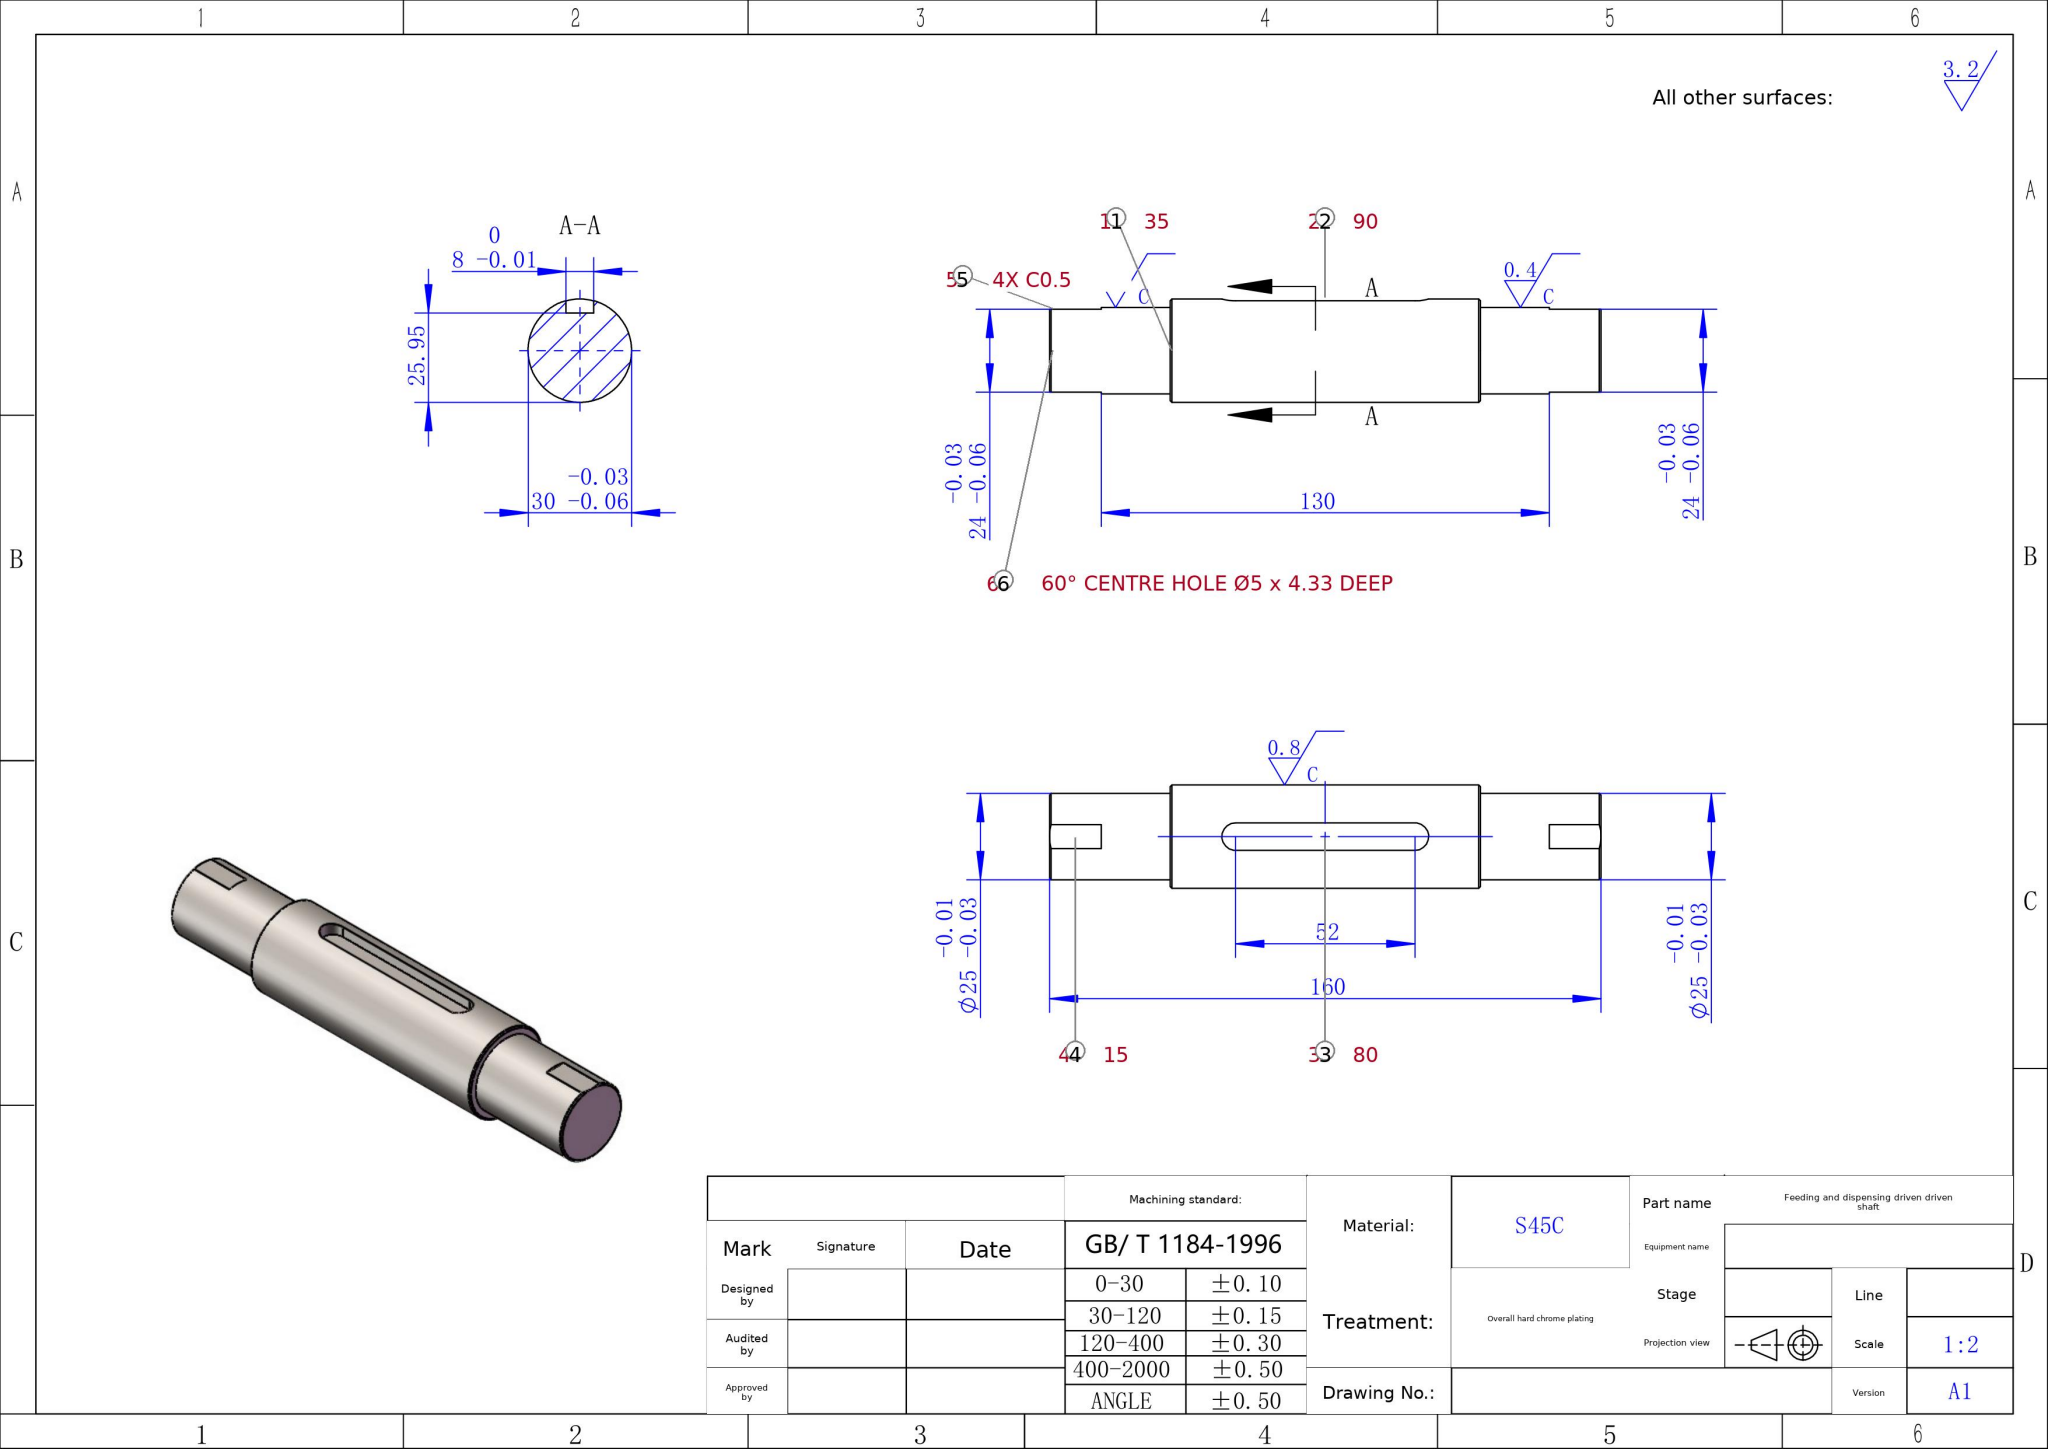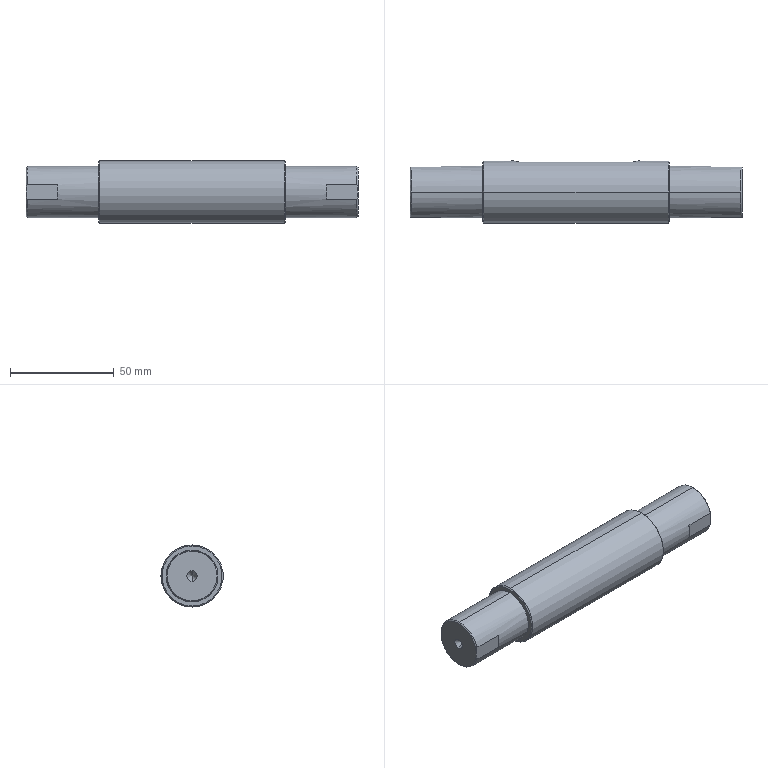Part | SolidWorks | mm | material S45C | 1 solid | 35 faces | box 160 x 30 x 30 mm | volume 95963 mm3 | plane 15 | cone 12 | cylinder 8 | commonest cylinder face diameters 25 x4 30 x2 8 x2
build123d program:
from build123d import *

# Parameters (mm, degrees)
CUT_EXTRUDE1_DEPTH      = 162.4
CUT_EXTRUDE1_DEPTH_BACK = 162.4
SKETCH2_W               = 15
SKETCH2_H               = 5.141
SKETCH2_H_2             = 5.357
CUT_EXTRUDE2_DEPTH      = 4.05


with BuildPart() as part:
    # Sketch1 → Revolve1 (revolve)
    with BuildSketch(Plane.XY, mode=Mode.PRIVATE) as revolve1_sk:
        Polygon((0, -2.5), (0, -12), (0.5, -12.5), (35, -12.5), (35, -14.5), (35.5, -15), (124.5, -15), (125, -14.5), (125, -12.5), (159.5, -12.5), (160, -12), (160, 0), (4.33, 0), align=None)
    revolve(revolve1_sk.sketch.rotate(Axis((0, 0, 0), (1, 0, 0)), 270), axis=Axis((0, 0, 0), (1, 0, 0)))

    # Sketch2 → Cut-Extrude1 (cut, two sides: drawn at the far end of the back side and taken through both)
    with BuildSketch(Plane.XY.offset(-CUT_EXTRUDE1_DEPTH_BACK)):
        with Locations((7.5, 14.571)):
            Rectangle(SKETCH2_W, SKETCH2_H)
        with Locations((152.5, 14.678)):
            Rectangle(SKETCH2_W, SKETCH2_H_2)
        with Locations((152.5, -14.678)):
            Rectangle(SKETCH2_W, SKETCH2_H_2)
        with Locations((7.5, -14.571)):
            Rectangle(SKETCH2_W, SKETCH2_H)
    extrude(amount=CUT_EXTRUDE1_DEPTH + CUT_EXTRUDE1_DEPTH_BACK, mode=Mode.SUBTRACT)

    # Sketch3 → Cut-Extrude2 (cut)
    with BuildSketch(Plane(origin=(0, 15, 0), x_dir=(1, 0, 0), z_dir=(0, 1, 0))):
        with BuildLine():
            Line((54, 4), (106, 4))
            ThreePointArc((106, 4), (110, 0), (106, -4))
            Line((106, -4), (54, -4))
            ThreePointArc((54, -4), (50, 0), (54, 4))
        make_face()
    extrude(amount=-CUT_EXTRUDE2_DEPTH, mode=Mode.SUBTRACT)


solid = part.part